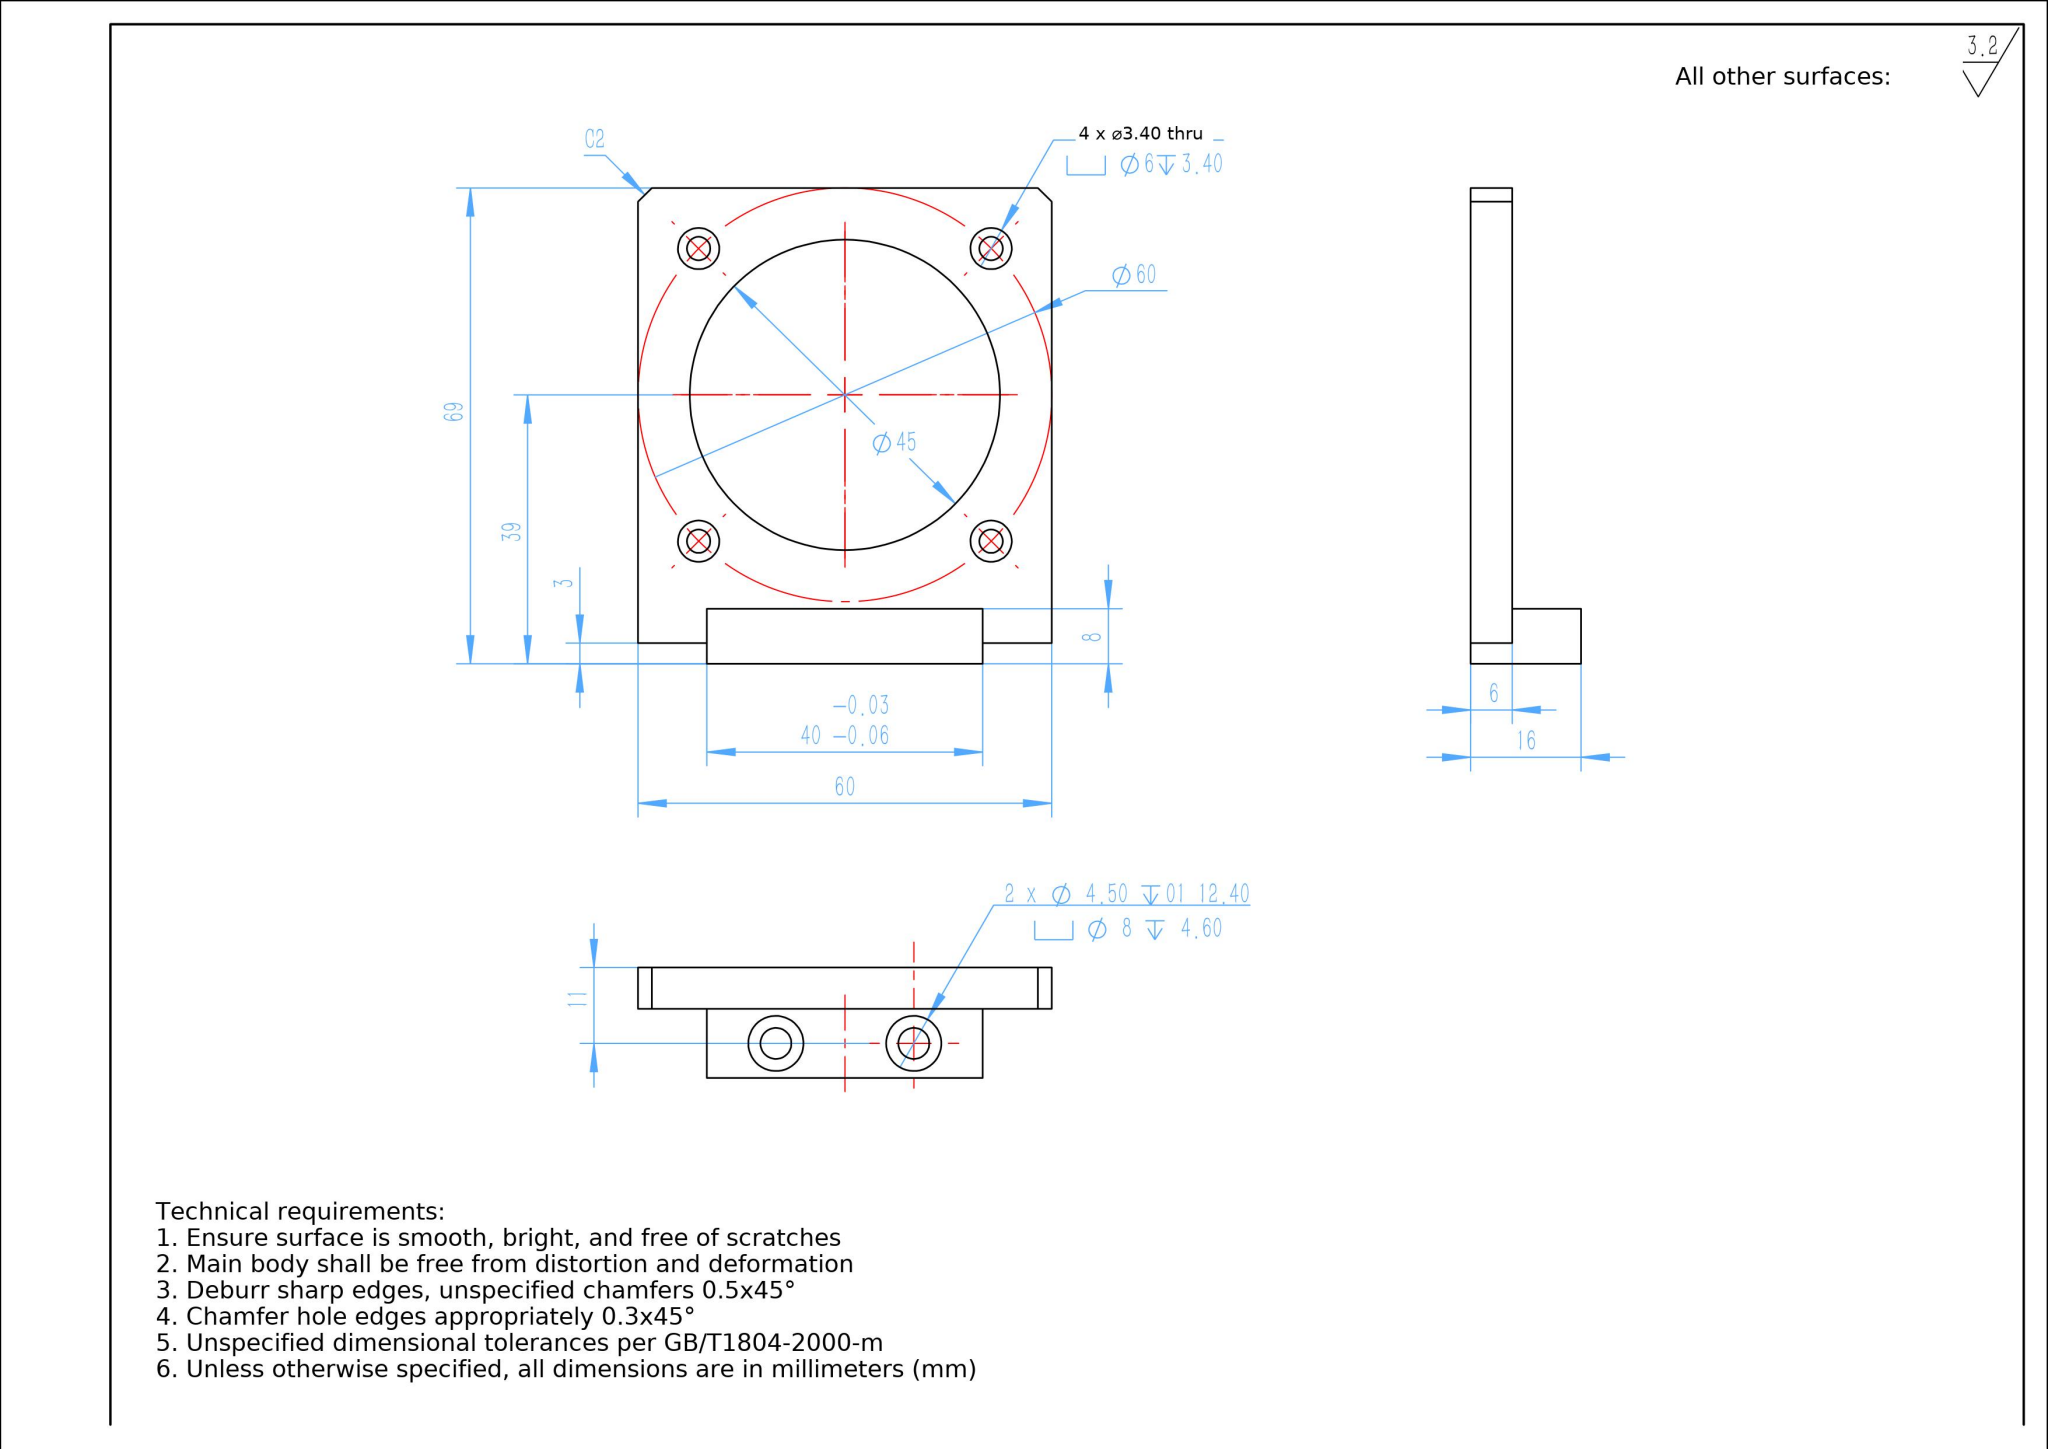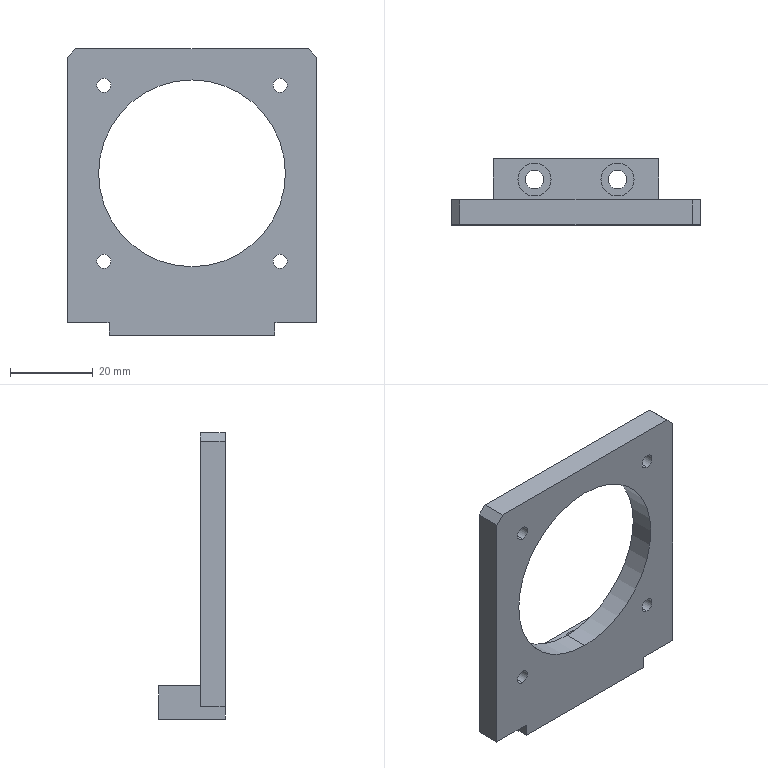Part | SolidWorks | mm | 1 solid | 50 faces | box 60 x 16 x 69 mm | volume 16886 mm3 | cylinder 28 | plane 20 | cone 2 | commonest cylinder face diameters 6 x8 3.4 x8 8 x4 4.5 x4 4.2 x2 45 x2
build123d program:
from build123d import *

# Parameters (mm, degrees)
SKETCH1_W                                         = 60
SKETCH1_H                                         = 66
BOSS_EXTRUDE1_DEPTH                               = 6
SKETCH3_W                                         = 40
SKETCH3_H                                         = 8
BOSS_EXTRUDE2_DEPTH                               = 16
SKETCH4_R                                         = 22.5
CUT_EXTRUDE1_DEPTH                                = 48.917
HOLE_SIZE_ACCORDING_TO_TYPE_2_HEX_SOC_D           = 3.4
HOLE_SIZE_ACCORDING_TO_TYPE_2_HEX_SOC_CBORE_D     = 6
HOLE_SIZE_ACCORDING_TO_TYPE_2_HEX_SOC_CBORE_DEPTH = 3.4
CHAMFER1_SIZE                                     = 2
M5_TAPPED_HOLE1_D                                 = 4.2
M5_TAPPED_HOLE1_DEPTH                             = 12.4
M5_TAPPED_HOLE1_TIP                               = 1.262
HOLE_SIZE_ACCORDING_TO_TYPE_2_HEX_2_D             = 4.5
HOLE_SIZE_ACCORDING_TO_TYPE_2_HEX_2_DEPTH         = 12.4
HOLE_SIZE_ACCORDING_TO_TYPE_2_HEX_2_CBORE_D       = 8
HOLE_SIZE_ACCORDING_TO_TYPE_2_HEX_2_CBORE_DEPTH   = 4.6
HOLE_SIZE_ACCORDING_TO_TYPE_2_HEX_2_TIP           = 1.352


with BuildPart() as part:
    # Sketch1 → Boss-Extrude1 (new body)
    with BuildSketch(Plane(origin=(0, 0, 0), x_dir=(1, 0, 0), z_dir=(0, 1, 0))):
        Rectangle(SKETCH1_W, SKETCH1_H)
    extrude(amount=-BOSS_EXTRUDE1_DEPTH)

    # Sketch3 → Boss-Extrude2 (add)
    with BuildSketch(Plane(origin=(0, -6, 0), x_dir=(1, 0, 0), z_dir=(0, 1, 0))):
        with Locations((0, 32)):
            Rectangle(SKETCH3_W, SKETCH3_H)
    extrude(amount=BOSS_EXTRUDE2_DEPTH)

    # Sketch4 → Cut-Extrude1 (cut, through all)
    with BuildSketch(Plane(origin=(0, 0, 0), x_dir=(1, 0, 0), z_dir=(0, 1, 0))):
        with Locations(Location((0, -3, 0), (0, 0, 270))):
            Circle(SKETCH4_R)
    extrude(amount=-CUT_EXTRUDE1_DEPTH, mode=Mode.SUBTRACT)

    # Hole Size _ according to_ Type 2 Hex Soc (through all)
    with Locations(Plane(origin=(0, 0, 0), x_dir=(1, 0, 0), z_dir=(0, 1, 0))):
        with Locations((-21.213, 18.213), (21.213, 18.213), (21.213, -24.213), (-21.213, -24.213)):
            CounterBoreHole(HOLE_SIZE_ACCORDING_TO_TYPE_2_HEX_SOC_D / 2, HOLE_SIZE_ACCORDING_TO_TYPE_2_HEX_SOC_CBORE_D / 2, HOLE_SIZE_ACCORDING_TO_TYPE_2_HEX_SOC_CBORE_DEPTH)

    # Chamfer1
    chamfer1_edges = [part.edges().sort_by_distance(p)[0] for p in [
        (30, -3, 33),
        (-30, -3, 33),
    ]]
    chamfer(chamfer1_edges, length=CHAMFER1_SIZE)

    # M5 Tapped Hole1
    with Locations(Plane(origin=(0, 0, -36), x_dir=(-1, 0, 0), z_dir=(0, 0, -1))):
        with Locations((0, -3)):
            Hole(M5_TAPPED_HOLE1_D / 2, depth=M5_TAPPED_HOLE1_DEPTH)
            with Locations((0, 0, -(M5_TAPPED_HOLE1_DEPTH + M5_TAPPED_HOLE1_TIP / 2))):  # 118° drill point
                Cone(0, M5_TAPPED_HOLE1_D / 2, M5_TAPPED_HOLE1_TIP, mode=Mode.SUBTRACT)

    # Hole Size _ according to_ Type 2 Hex 2
    with Locations(Plane.XY.offset(-28)):
        with Locations((-10, 5), (10, 5)):
            CounterBoreHole(HOLE_SIZE_ACCORDING_TO_TYPE_2_HEX_2_D / 2, HOLE_SIZE_ACCORDING_TO_TYPE_2_HEX_2_CBORE_D / 2, HOLE_SIZE_ACCORDING_TO_TYPE_2_HEX_2_CBORE_DEPTH, depth=HOLE_SIZE_ACCORDING_TO_TYPE_2_HEX_2_DEPTH)
            with Locations((0, 0, -(HOLE_SIZE_ACCORDING_TO_TYPE_2_HEX_2_DEPTH + HOLE_SIZE_ACCORDING_TO_TYPE_2_HEX_2_TIP / 2))):  # 118° drill point
                Cone(0, HOLE_SIZE_ACCORDING_TO_TYPE_2_HEX_2_D / 2, HOLE_SIZE_ACCORDING_TO_TYPE_2_HEX_2_TIP, mode=Mode.SUBTRACT)


solid = part.part